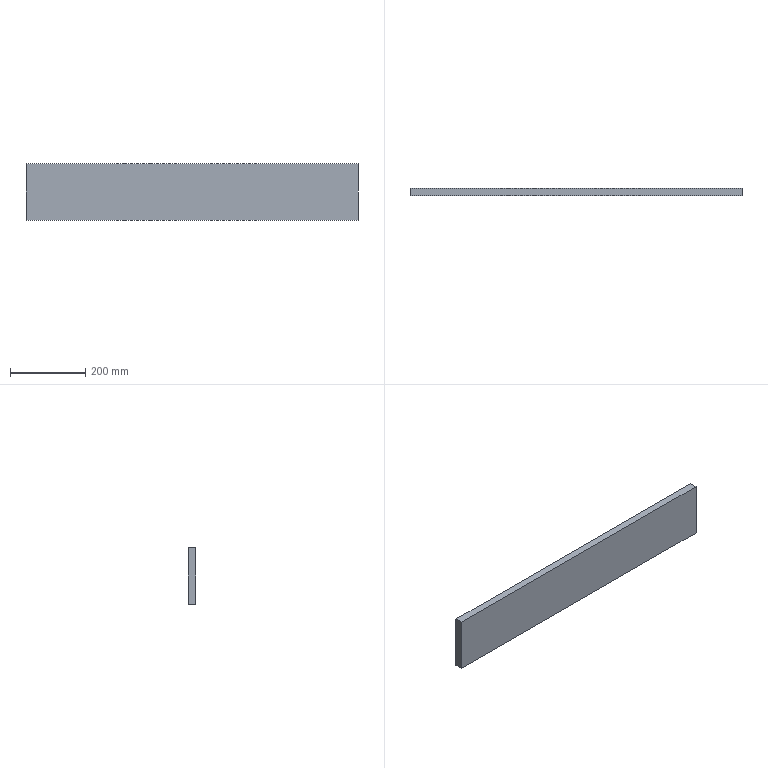Component | SolidWorks | JF21-80.1-1-3(_)-1-SOLID38-1 | 1 solid | 6 faces | box 880 x 20 x 150 mm | volume 2640000 mm3 | plane 6
STEP:
#1=COLOUR_RGB('',0.7922,0.8196,0.9333);
#2=FILL_AREA_STYLE_COLOUR('',#1);
#3=FILL_AREA_STYLE('',(#2));
#4=SURFACE_STYLE_FILL_AREA(#3);
#5=SURFACE_SIDE_STYLE('',(#4));
#6=SURFACE_STYLE_USAGE(.BOTH.,#5);
#7=PRESENTATION_STYLE_ASSIGNMENT((#6));
#8=CARTESIAN_POINT('',(-17.323,-88.583,29.528));
#9=VERTEX_POINT('',#8);
#10=CARTESIAN_POINT('',(-17.323,-88.583,23.622));
#11=VERTEX_POINT('',#10);
#12=CARTESIAN_POINT('',(-17.323,-88.583,23.622));
#13=DIRECTION('',(0.,0.,-1.));
#14=VECTOR('',#13,39.37);
#15=LINE('',#12,#14);
#16=EDGE_CURVE('',#9,#11,#15,.T.);
#17=ORIENTED_EDGE('',*,*,#16,.T.);
#18=CARTESIAN_POINT('',(-17.323,-89.37,23.622));
#19=VERTEX_POINT('',#18);
#20=CARTESIAN_POINT('',(-17.323,-89.37,23.622));
#21=DIRECTION('',(0.,1.,0.));
#22=VECTOR('',#21,39.37);
#23=LINE('',#20,#22);
#24=EDGE_CURVE('',#19,#11,#23,.T.);
#25=ORIENTED_EDGE('',*,*,#24,.F.);
#26=CARTESIAN_POINT('',(-17.323,-89.37,29.528));
#27=VERTEX_POINT('',#26);
#28=CARTESIAN_POINT('',(-17.323,-89.37,23.622));
#29=DIRECTION('',(0.,0.,-1.));
#30=VECTOR('',#29,39.37);
#31=LINE('',#28,#30);
#32=EDGE_CURVE('',#27,#19,#31,.T.);
#33=ORIENTED_EDGE('',*,*,#32,.F.);
#34=CARTESIAN_POINT('',(-17.323,-89.37,29.528));
#35=DIRECTION('',(0.,1.,0.));
#36=VECTOR('',#35,39.37);
#37=LINE('',#34,#36);
#38=EDGE_CURVE('',#27,#9,#37,.T.);
#39=ORIENTED_EDGE('',*,*,#38,.T.);
#40=EDGE_LOOP('',(#17,#25,#33,#39));
#41=FACE_OUTER_BOUND('',#40,.T.);
#42=CARTESIAN_POINT('',(-17.323,-89.37,23.622));
#43=DIRECTION('',(1.,0.,0.));
#44=DIRECTION('',(0.,0.,1.));
#45=AXIS2_PLACEMENT_3D('',#42,#43,#44);
#46=PLANE('',#45);
#47=ADVANCED_FACE('',(#41),#46,.F.);
#48=CARTESIAN_POINT('',(17.323,-88.583,23.622));
#49=VERTEX_POINT('',#48);
#50=CARTESIAN_POINT('',(-17.323,-88.583,23.622));
#51=DIRECTION('',(1.,0.,0.));
#52=VECTOR('',#51,39.37);
#53=LINE('',#50,#52);
#54=EDGE_CURVE('',#11,#49,#53,.T.);
#55=ORIENTED_EDGE('',*,*,#54,.T.);
#56=CARTESIAN_POINT('',(17.323,-89.37,23.622));
#57=VERTEX_POINT('',#56);
#58=CARTESIAN_POINT('',(17.323,-89.37,23.622));
#59=DIRECTION('',(0.,1.,0.));
#60=VECTOR('',#59,39.37);
#61=LINE('',#58,#60);
#62=EDGE_CURVE('',#57,#49,#61,.T.);
#63=ORIENTED_EDGE('',*,*,#62,.F.);
#64=CARTESIAN_POINT('',(-17.323,-89.37,23.622));
#65=DIRECTION('',(1.,0.,0.));
#66=VECTOR('',#65,39.37);
#67=LINE('',#64,#66);
#68=EDGE_CURVE('',#19,#57,#67,.T.);
#69=ORIENTED_EDGE('',*,*,#68,.F.);
#70=ORIENTED_EDGE('',*,*,#24,.T.);
#71=EDGE_LOOP('',(#55,#63,#69,#70));
#72=FACE_OUTER_BOUND('',#71,.T.);
#73=CARTESIAN_POINT('',(-17.323,-89.37,23.622));
#74=DIRECTION('',(0.,0.,1.));
#75=DIRECTION('',(-1.,0.,0.));
#76=AXIS2_PLACEMENT_3D('',#73,#74,#75);
#77=PLANE('',#76);
#78=ADVANCED_FACE('',(#72),#77,.F.);
#79=CARTESIAN_POINT('',(17.323,-88.583,29.528));
#80=VERTEX_POINT('',#79);
#81=CARTESIAN_POINT('',(17.323,-88.583,23.622));
#82=DIRECTION('',(0.,0.,1.));
#83=VECTOR('',#82,39.37);
#84=LINE('',#81,#83);
#85=EDGE_CURVE('',#49,#80,#84,.T.);
#86=ORIENTED_EDGE('',*,*,#85,.T.);
#87=CARTESIAN_POINT('',(17.323,-89.37,29.528));
#88=VERTEX_POINT('',#87);
#89=CARTESIAN_POINT('',(17.323,-89.37,29.528));
#90=DIRECTION('',(0.,1.,0.));
#91=VECTOR('',#90,39.37);
#92=LINE('',#89,#91);
#93=EDGE_CURVE('',#88,#80,#92,.T.);
#94=ORIENTED_EDGE('',*,*,#93,.F.);
#95=CARTESIAN_POINT('',(17.323,-89.37,23.622));
#96=DIRECTION('',(0.,0.,1.));
#97=VECTOR('',#96,39.37);
#98=LINE('',#95,#97);
#99=EDGE_CURVE('',#57,#88,#98,.T.);
#100=ORIENTED_EDGE('',*,*,#99,.F.);
#101=ORIENTED_EDGE('',*,*,#62,.T.);
#102=EDGE_LOOP('',(#86,#94,#100,#101));
#103=FACE_OUTER_BOUND('',#102,.T.);
#104=CARTESIAN_POINT('',(17.323,-89.37,23.622));
#105=DIRECTION('',(-1.,0.,0.));
#106=DIRECTION('',(0.,0.,-1.));
#107=AXIS2_PLACEMENT_3D('',#104,#105,#106);
#108=PLANE('',#107);
#109=ADVANCED_FACE('',(#103),#108,.F.);
#110=CARTESIAN_POINT('',(-17.323,-88.583,29.528));
#111=DIRECTION('',(-1.,0.,0.));
#112=VECTOR('',#111,39.37);
#113=LINE('',#110,#112);
#114=EDGE_CURVE('',#80,#9,#113,.T.);
#115=ORIENTED_EDGE('',*,*,#114,.T.);
#116=ORIENTED_EDGE('',*,*,#38,.F.);
#117=CARTESIAN_POINT('',(-17.323,-89.37,29.528));
#118=DIRECTION('',(-1.,0.,0.));
#119=VECTOR('',#118,39.37);
#120=LINE('',#117,#119);
#121=EDGE_CURVE('',#88,#27,#120,.T.);
#122=ORIENTED_EDGE('',*,*,#121,.F.);
#123=ORIENTED_EDGE('',*,*,#93,.T.);
#124=EDGE_LOOP('',(#115,#116,#122,#123));
#125=FACE_OUTER_BOUND('',#124,.T.);
#126=CARTESIAN_POINT('',(-17.323,-89.37,29.528));
#127=DIRECTION('',(0.,0.,-1.));
#128=DIRECTION('',(1.,0.,0.));
#129=AXIS2_PLACEMENT_3D('',#126,#127,#128);
#130=PLANE('',#129);
#131=ADVANCED_FACE('',(#125),#130,.F.);
#132=ORIENTED_EDGE('',*,*,#32,.T.);
#133=ORIENTED_EDGE('',*,*,#68,.T.);
#134=ORIENTED_EDGE('',*,*,#99,.T.);
#135=ORIENTED_EDGE('',*,*,#121,.T.);
#136=EDGE_LOOP('',(#132,#133,#134,#135));
#137=FACE_OUTER_BOUND('',#136,.T.);
#138=CARTESIAN_POINT('',(-17.323,-89.37,29.528));
#139=DIRECTION('',(0.,1.,0.));
#140=DIRECTION('',(0.,0.,-1.));
#141=AXIS2_PLACEMENT_3D('',#138,#139,#140);
#142=PLANE('',#141);
#143=ADVANCED_FACE('',(#137),#142,.F.);
#144=ORIENTED_EDGE('',*,*,#16,.F.);
#145=ORIENTED_EDGE('',*,*,#114,.F.);
#146=ORIENTED_EDGE('',*,*,#85,.F.);
#147=ORIENTED_EDGE('',*,*,#54,.F.);
#148=EDGE_LOOP('',(#144,#145,#146,#147));
#149=FACE_OUTER_BOUND('',#148,.T.);
#150=CARTESIAN_POINT('',(-17.323,-88.583,29.528));
#151=DIRECTION('',(0.,1.,0.));
#152=DIRECTION('',(0.,0.,-1.));
#153=AXIS2_PLACEMENT_3D('',#150,#151,#152);
#154=PLANE('',#153);
#155=ADVANCED_FACE('',(#149),#154,.T.);
#156=CLOSED_SHELL('',(#47,#78,#109,#131,#143,#155));
#157=MANIFOLD_SOLID_BREP('',#156);
#158=STYLED_ITEM('',(#7),#157);
#159=(LENGTH_UNIT()NAMED_UNIT(*)SI_UNIT($,.METRE.));
#160=LENGTH_MEASURE_WITH_UNIT(LENGTH_MEASURE(0.0254),#159);
#161=DIMENSIONAL_EXPONENTS(1.,0.,0.,0.,0.,0.,0.);
#162=(CONVERSION_BASED_UNIT('',#160)LENGTH_UNIT()NAMED_UNIT(#161));
#163=UNCERTAINTY_MEASURE_WITH_UNIT(LENGTH_MEASURE(0.00001),#162,'','');
#164=(NAMED_UNIT(*)PLANE_ANGLE_UNIT()SI_UNIT($,.RADIAN.));
#165=(NAMED_UNIT(*)SI_UNIT($,.STERADIAN.)SOLID_ANGLE_UNIT());
#166=(GEOMETRIC_REPRESENTATION_CONTEXT(3)GLOBAL_UNCERTAINTY_ASSIGNED_CONTEXT((#163))GLOBAL_UNIT_ASSIGNED_CONTEXT((#162,#164,#165))REPRESENTATION_CONTEXT('',''));
#167=MECHANICAL_DESIGN_GEOMETRIC_PRESENTATION_REPRESENTATION('',(#158),#166);
#168=PRESENTATION_LAYER_ASSIGNMENT('','',(#158));
#169=CARTESIAN_POINT('',(0.,0.,0.));
#170=DIRECTION('',(0.,0.,1.));
#171=DIRECTION('',(1.,0.,0.));
#172=AXIS2_PLACEMENT_3D('',#169,#170,#171);
#173=(LENGTH_UNIT()NAMED_UNIT(*)SI_UNIT($,.METRE.));
#174=LENGTH_MEASURE_WITH_UNIT(LENGTH_MEASURE(0.0254),#173);
#175=DIMENSIONAL_EXPONENTS(1.,0.,0.,0.,0.,0.,0.);
#176=(CONVERSION_BASED_UNIT('',#174)LENGTH_UNIT()NAMED_UNIT(#175));
#177=UNCERTAINTY_MEASURE_WITH_UNIT(LENGTH_MEASURE(0.00001),#176,'','');
#178=(NAMED_UNIT(*)PLANE_ANGLE_UNIT()SI_UNIT($,.RADIAN.));
#179=(NAMED_UNIT(*)SI_UNIT($,.STERADIAN.)SOLID_ANGLE_UNIT());
#180=(GEOMETRIC_REPRESENTATION_CONTEXT(3)GLOBAL_UNCERTAINTY_ASSIGNED_CONTEXT((#177))GLOBAL_UNIT_ASSIGNED_CONTEXT((#176,#178,#179))REPRESENTATION_CONTEXT('',''));
#181=ADVANCED_BREP_SHAPE_REPRESENTATION('',(#157,#172),#180);